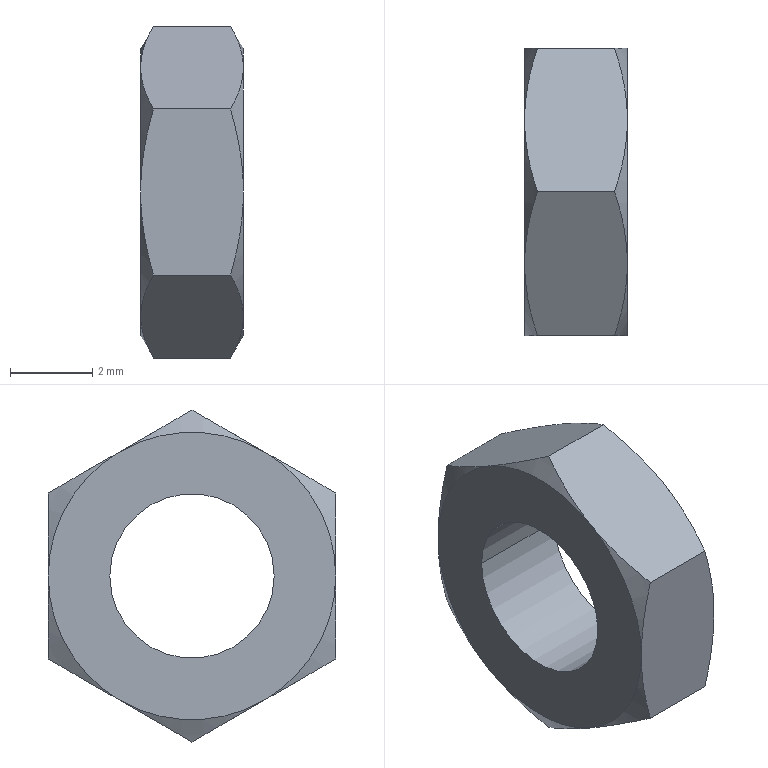Component | SolidWorks | MI10x10U(0)+()-1_MI10-M4x0_7 - Nut-2 | 1 solid | 22 faces | box 2.5 x 7 x 8.08 mm | volume 74 mm3 | cone 12 | plane 8 | cylinder 2 | commonest cylinder face diameters 4 x2
build123d program:
from build123d import *

# Parameters (mm, degrees)
SKETCH2_W                        = 14
SKETCH2_H                        = 14
CUT_EXTRUDE1_DEPTH               = 5
SKETCH1_R                        = 2
M4_THREAD_MAJOR_DIA_RELIEF_DEPTH = 6.902


with BuildPart() as part:
    # Sketch1_2 → Revolve1 (revolve)
    with BuildSketch(Plane.XY, mode=Mode.PRIVATE) as revolve1_sk:
        Polygon((0, 0), (0, 3.5), (0.4041, 4.2), (2.096, 4.2), (2.5, 3.5), (2.5, 0), align=None)
    revolve(revolve1_sk.sketch.rotate(Axis((2.5, 0, 0), (-1, 0, 0)), 270), axis=Axis((2.5, 0, 0), (-1, 0, 0)))

    # Sketch2 → Cut-Extrude1 (cut)
    with BuildSketch(Plane(origin=(0, 0, 0), x_dir=(0, 0, -1), z_dir=(1, 0, 0))):
        Rectangle(SKETCH2_W, SKETCH2_H)
        Polygon((-3.5, -2.021), (0, -4.041), (3.5, -2.021), (3.5, 2.021), (0, 4.041), (-3.5, 2.021), align=None, mode=Mode.SUBTRACT)
    extrude(amount=CUT_EXTRUDE1_DEPTH, mode=Mode.SUBTRACT)

    # Sketch3 → Cut-Revolve1 (revolve, cut)
    with BuildSketch(Plane.XY, mode=Mode.PRIVATE) as cut_revolve1_sk:
        Polygon((0, 0), (0, 2), (0.379, 1.621), (2.121, 1.621), (2.5, 2), (2.5, 0), align=None)
    revolve(cut_revolve1_sk.sketch.rotate(Axis((2.5, 0, 0), (-1, 0, 0)), 270), axis=Axis((2.5, 0, 0), (-1, 0, 0)), mode=Mode.SUBTRACT)

    # Sketch1 → M4 thread major-dia relief (cut, through all)
    with BuildSketch(Plane.ZY):
        Circle(SKETCH1_R)
    extrude(amount=-M4_THREAD_MAJOR_DIA_RELIEF_DEPTH, mode=Mode.SUBTRACT)


solid = part.part

# Placed as in the assembly
solid = solid.moved(Location((-0.994, 30.452, 72.77), (90, 0, 0)))
STEP:
#1=COLOUR_RGB('',0.7922,0.8196,0.9333);
#2=FILL_AREA_STYLE_COLOUR('',#1);
#3=FILL_AREA_STYLE('',(#2));
#4=SURFACE_STYLE_FILL_AREA(#3);
#5=SURFACE_SIDE_STYLE('',(#4));
#6=SURFACE_STYLE_USAGE(.BOTH.,#5);
#7=PRESENTATION_STYLE_ASSIGNMENT((#6));
#8=CARTESIAN_POINT('',(-0.03913,1.12,2.865));
#9=VERTEX_POINT('',#8);
#10=CARTESIAN_POINT('',(-0.03913,1.278,2.865));
#11=VERTEX_POINT('',#10);
#12=CARTESIAN_POINT('',(-0.03913,1.199,2.865));
#13=DIRECTION('',(1.,-0.,-0.));
#14=DIRECTION('',(0.,1.,0.));
#15=AXIS2_PLACEMENT_3D('',#12,#13,#14);
#16=CIRCLE('',#15,0.07874);
#17=EDGE_CURVE('',#9,#11,#16,.T.);
#18=ORIENTED_EDGE('',*,*,#17,.F.);
#19=CARTESIAN_POINT('',(0.05929,1.12,2.865));
#20=VERTEX_POINT('',#19);
#21=CARTESIAN_POINT('',(-0.03913,1.12,2.865));
#22=DIRECTION('',(1.,-0.,-0.));
#23=VECTOR('',#22,39.37);
#24=LINE('',#21,#23);
#25=EDGE_CURVE('',#9,#20,#24,.T.);
#26=ORIENTED_EDGE('',*,*,#25,.T.);
#27=CARTESIAN_POINT('',(0.05929,1.278,2.865));
#28=VERTEX_POINT('',#27);
#29=CARTESIAN_POINT('',(0.05929,1.199,2.865));
#30=DIRECTION('',(1.,-0.,-0.));
#31=DIRECTION('',(0.,1.,0.));
#32=AXIS2_PLACEMENT_3D('',#29,#30,#31);
#33=CIRCLE('',#32,0.07874);
#34=EDGE_CURVE('',#20,#28,#33,.T.);
#35=ORIENTED_EDGE('',*,*,#34,.T.);
#36=CARTESIAN_POINT('',(-0.03913,1.278,2.865));
#37=DIRECTION('',(1.,-0.,-0.));
#38=VECTOR('',#37,39.37);
#39=LINE('',#36,#38);
#40=EDGE_CURVE('',#11,#28,#39,.T.);
#41=ORIENTED_EDGE('',*,*,#40,.F.);
#42=EDGE_LOOP('',(#18,#26,#35,#41));
#43=FACE_OUTER_BOUND('',#42,.T.);
#44=CARTESIAN_POINT('',(-0.03913,1.199,2.865));
#45=DIRECTION('',(1.,-0.,-0.));
#46=DIRECTION('',(0.,1.,0.));
#47=AXIS2_PLACEMENT_3D('',#44,#45,#46);
#48=CYLINDRICAL_SURFACE('',#47,0.07874);
#49=ADVANCED_FACE('',(#43),#48,.F.);
#50=CARTESIAN_POINT('',(0.05929,1.061,2.865));
#51=VERTEX_POINT('',#50);
#52=CARTESIAN_POINT('',(0.04698,1.061,2.785));
#53=VERTEX_POINT('',#52);
#54=CARTESIAN_POINT('',(0.05929,1.061,2.865));
#55=CARTESIAN_POINT('',(0.05929,1.061,2.852));
#56=CARTESIAN_POINT('',(0.05814,1.061,2.838));
#57=CARTESIAN_POINT('',(0.05385,1.061,2.812));
#58=CARTESIAN_POINT('',(0.05072,1.061,2.798));
#59=CARTESIAN_POINT('',(0.04698,1.061,2.785));
#60=B_SPLINE_CURVE_WITH_KNOTS('',3,(#54,#55,#56,#57,#58,#59),.UNSPECIFIED.,.F.,.F.,(4,2,4),(0.01092,0.01194,0.01297),.UNSPECIFIED.);
#61=EDGE_CURVE('',#51,#53,#60,.T.);
#62=ORIENTED_EDGE('',*,*,#61,.T.);
#63=CARTESIAN_POINT('',(0.05929,1.13,2.746));
#64=VERTEX_POINT('',#63);
#65=CARTESIAN_POINT('',(0.04698,1.061,2.785));
#66=CARTESIAN_POINT('',(0.0545,1.084,2.772));
#67=CARTESIAN_POINT('',(0.05929,1.107,2.759));
#68=CARTESIAN_POINT('',(0.05929,1.13,2.746));
#69=B_SPLINE_CURVE_WITH_KNOTS('',3,(#65,#66,#67,#68),.UNSPECIFIED.,.F.,.F.,(4,4),(0.00000024,0.002045),.UNSPECIFIED.);
#70=EDGE_CURVE('',#53,#64,#69,.T.);
#71=ORIENTED_EDGE('',*,*,#70,.T.);
#72=CARTESIAN_POINT('',(0.05929,1.199,2.865));
#73=DIRECTION('',(1.,-0.,-0.));
#74=DIRECTION('',(0.,1.,0.));
#75=AXIS2_PLACEMENT_3D('',#72,#73,#74);
#76=CIRCLE('',#75,0.1378);
#77=EDGE_CURVE('',#51,#64,#76,.T.);
#78=ORIENTED_EDGE('',*,*,#77,.F.);
#79=EDGE_LOOP('',(#62,#71,#78));
#80=FACE_OUTER_BOUND('',#79,.T.);
#81=CARTESIAN_POINT('',(0.04338,1.199,2.865));
#82=DIRECTION('',(-1.,0.,0.));
#83=DIRECTION('',(-0.,-1.,0.));
#84=AXIS2_PLACEMENT_3D('',#81,#82,#83);
#85=CONICAL_SURFACE('',#84,0.1654,1.047);
#86=ADVANCED_FACE('',(#80),#85,.T.);
#87=CARTESIAN_POINT('',(0.05929,1.268,2.746));
#88=VERTEX_POINT('',#87);
#89=CARTESIAN_POINT('',(0.05929,1.199,2.865));
#90=DIRECTION('',(1.,-0.,-0.));
#91=DIRECTION('',(0.,1.,0.));
#92=AXIS2_PLACEMENT_3D('',#89,#90,#91);
#93=CIRCLE('',#92,0.1378);
#94=EDGE_CURVE('',#64,#88,#93,.T.);
#95=ORIENTED_EDGE('',*,*,#94,.F.);
#96=CARTESIAN_POINT('',(0.04698,1.199,2.706));
#97=VERTEX_POINT('',#96);
#98=CARTESIAN_POINT('',(0.05929,1.13,2.746));
#99=CARTESIAN_POINT('',(0.05929,1.142,2.739));
#100=CARTESIAN_POINT('',(0.05811,1.153,2.732));
#101=CARTESIAN_POINT('',(0.05382,1.176,2.719));
#102=CARTESIAN_POINT('',(0.05073,1.188,2.712));
#103=CARTESIAN_POINT('',(0.04698,1.199,2.706));
#104=B_SPLINE_CURVE_WITH_KNOTS('',3,(#98,#99,#100,#101,#102,#103),.UNSPECIFIED.,.F.,.F.,(4,2,4),(0.002045,0.003063,0.004082),.UNSPECIFIED.);
#105=EDGE_CURVE('',#64,#97,#104,.T.);
#106=ORIENTED_EDGE('',*,*,#105,.T.);
#107=CARTESIAN_POINT('',(0.04698,1.199,2.706));
#108=CARTESIAN_POINT('',(0.0545,1.221,2.719));
#109=CARTESIAN_POINT('',(0.05929,1.244,2.732));
#110=CARTESIAN_POINT('',(0.05929,1.268,2.746));
#111=B_SPLINE_CURVE_WITH_KNOTS('',3,(#107,#108,#109,#110),.UNSPECIFIED.,.F.,.F.,(4,4),(0.00000024,0.002045),.UNSPECIFIED.);
#112=EDGE_CURVE('',#97,#88,#111,.T.);
#113=ORIENTED_EDGE('',*,*,#112,.T.);
#114=EDGE_LOOP('',(#95,#106,#113));
#115=FACE_OUTER_BOUND('',#114,.T.);
#116=CARTESIAN_POINT('',(0.04338,1.199,2.865));
#117=DIRECTION('',(-1.,0.,0.));
#118=DIRECTION('',(-0.,-1.,0.));
#119=AXIS2_PLACEMENT_3D('',#116,#117,#118);
#120=CONICAL_SURFACE('',#119,0.1654,1.047);
#121=ADVANCED_FACE('',(#115),#120,.T.);
#122=CARTESIAN_POINT('',(0.05929,1.337,2.865));
#123=VERTEX_POINT('',#122);
#124=CARTESIAN_POINT('',(0.05929,1.199,2.865));
#125=DIRECTION('',(1.,-0.,-0.));
#126=DIRECTION('',(0.,1.,0.));
#127=AXIS2_PLACEMENT_3D('',#124,#125,#126);
#128=CIRCLE('',#127,0.1378);
#129=EDGE_CURVE('',#88,#123,#128,.T.);
#130=ORIENTED_EDGE('',*,*,#129,.F.);
#131=CARTESIAN_POINT('',(0.04698,1.337,2.785));
#132=VERTEX_POINT('',#131);
#133=CARTESIAN_POINT('',(0.05929,1.268,2.746));
#134=CARTESIAN_POINT('',(0.05929,1.28,2.752));
#135=CARTESIAN_POINT('',(0.05811,1.291,2.759));
#136=CARTESIAN_POINT('',(0.05382,1.314,2.772));
#137=CARTESIAN_POINT('',(0.05073,1.325,2.779));
#138=CARTESIAN_POINT('',(0.04698,1.337,2.785));
#139=B_SPLINE_CURVE_WITH_KNOTS('',3,(#133,#134,#135,#136,#137,#138),.UNSPECIFIED.,.F.,.F.,(4,2,4),(0.002045,0.003063,0.004082),.UNSPECIFIED.);
#140=EDGE_CURVE('',#88,#132,#139,.T.);
#141=ORIENTED_EDGE('',*,*,#140,.T.);
#142=CARTESIAN_POINT('',(0.04698,1.337,2.785));
#143=CARTESIAN_POINT('',(0.05072,1.337,2.798));
#144=CARTESIAN_POINT('',(0.05385,1.337,2.812));
#145=CARTESIAN_POINT('',(0.05814,1.337,2.838));
#146=CARTESIAN_POINT('',(0.05929,1.337,2.852));
#147=CARTESIAN_POINT('',(0.05929,1.337,2.865));
#148=B_SPLINE_CURVE_WITH_KNOTS('',3,(#142,#143,#144,#145,#146,#147),.UNSPECIFIED.,.F.,.F.,(4,2,4),(0.003619,0.004642,0.005664),.UNSPECIFIED.);
#149=EDGE_CURVE('',#132,#123,#148,.T.);
#150=ORIENTED_EDGE('',*,*,#149,.T.);
#151=EDGE_LOOP('',(#130,#141,#150));
#152=FACE_OUTER_BOUND('',#151,.T.);
#153=CARTESIAN_POINT('',(0.04338,1.199,2.865));
#154=DIRECTION('',(-1.,0.,0.));
#155=DIRECTION('',(-0.,-1.,0.));
#156=AXIS2_PLACEMENT_3D('',#153,#154,#155);
#157=CONICAL_SURFACE('',#156,0.1654,1.047);
#158=ADVANCED_FACE('',(#152),#157,.T.);
#159=CARTESIAN_POINT('',(0.05929,1.13,2.984));
#160=VERTEX_POINT('',#159);
#161=CARTESIAN_POINT('',(0.04698,1.061,2.945));
#162=VERTEX_POINT('',#161);
#163=CARTESIAN_POINT('',(0.05929,1.13,2.984));
#164=CARTESIAN_POINT('',(0.05929,1.118,2.978));
#165=CARTESIAN_POINT('',(0.05811,1.107,2.971));
#166=CARTESIAN_POINT('',(0.05382,1.084,2.958));
#167=CARTESIAN_POINT('',(0.05073,1.072,2.951));
#168=CARTESIAN_POINT('',(0.04698,1.061,2.945));
#169=B_SPLINE_CURVE_WITH_KNOTS('',3,(#163,#164,#165,#166,#167,#168),.UNSPECIFIED.,.F.,.F.,(4,2,4),(0.002045,0.003063,0.004082),.UNSPECIFIED.);
#170=EDGE_CURVE('',#160,#162,#169,.T.);
#171=ORIENTED_EDGE('',*,*,#170,.T.);
#172=CARTESIAN_POINT('',(0.04698,1.061,2.945));
#173=CARTESIAN_POINT('',(0.0507,1.061,2.932));
#174=CARTESIAN_POINT('',(0.05379,1.061,2.919));
#175=CARTESIAN_POINT('',(0.0581,1.061,2.892));
#176=CARTESIAN_POINT('',(0.05929,1.061,2.878));
#177=CARTESIAN_POINT('',(0.05929,1.061,2.865));
#178=B_SPLINE_CURVE_WITH_KNOTS('',3,(#172,#173,#174,#175,#176,#177),.UNSPECIFIED.,.F.,.F.,(4,2,4),(0.008871,0.009895,0.01092),.UNSPECIFIED.);
#179=EDGE_CURVE('',#162,#51,#178,.T.);
#180=ORIENTED_EDGE('',*,*,#179,.T.);
#181=CARTESIAN_POINT('',(0.05929,1.199,2.865));
#182=DIRECTION('',(1.,-0.,-0.));
#183=DIRECTION('',(0.,1.,0.));
#184=AXIS2_PLACEMENT_3D('',#181,#182,#183);
#185=CIRCLE('',#184,0.1378);
#186=EDGE_CURVE('',#160,#51,#185,.T.);
#187=ORIENTED_EDGE('',*,*,#186,.F.);
#188=EDGE_LOOP('',(#171,#180,#187));
#189=FACE_OUTER_BOUND('',#188,.T.);
#190=CARTESIAN_POINT('',(0.04338,1.199,2.865));
#191=DIRECTION('',(-1.,0.,0.));
#192=DIRECTION('',(-0.,-1.,0.));
#193=AXIS2_PLACEMENT_3D('',#190,#191,#192);
#194=CONICAL_SURFACE('',#193,0.1654,1.047);
#195=ADVANCED_FACE('',(#189),#194,.T.);
#196=CARTESIAN_POINT('',(0.05929,1.268,2.984));
#197=VERTEX_POINT('',#196);
#198=CARTESIAN_POINT('',(0.05929,1.199,2.865));
#199=DIRECTION('',(1.,-0.,-0.));
#200=DIRECTION('',(0.,1.,0.));
#201=AXIS2_PLACEMENT_3D('',#198,#199,#200);
#202=CIRCLE('',#201,0.1378);
#203=EDGE_CURVE('',#123,#197,#202,.T.);
#204=ORIENTED_EDGE('',*,*,#203,.F.);
#205=CARTESIAN_POINT('',(0.04698,1.337,2.945));
#206=VERTEX_POINT('',#205);
#207=CARTESIAN_POINT('',(0.05929,1.337,2.865));
#208=CARTESIAN_POINT('',(0.05929,1.337,2.878));
#209=CARTESIAN_POINT('',(0.0581,1.337,2.892));
#210=CARTESIAN_POINT('',(0.05379,1.337,2.919));
#211=CARTESIAN_POINT('',(0.0507,1.337,2.932));
#212=CARTESIAN_POINT('',(0.04698,1.337,2.945));
#213=B_SPLINE_CURVE_WITH_KNOTS('',3,(#207,#208,#209,#210,#211,#212),.UNSPECIFIED.,.F.,.F.,(4,2,4),(0.005664,0.006687,0.007709),.UNSPECIFIED.);
#214=EDGE_CURVE('',#123,#206,#213,.T.);
#215=ORIENTED_EDGE('',*,*,#214,.T.);
#216=CARTESIAN_POINT('',(0.04698,1.337,2.945));
#217=CARTESIAN_POINT('',(0.0545,1.314,2.958));
#218=CARTESIAN_POINT('',(0.05929,1.291,2.971));
#219=CARTESIAN_POINT('',(0.05929,1.268,2.984));
#220=B_SPLINE_CURVE_WITH_KNOTS('',3,(#216,#217,#218,#219),.UNSPECIFIED.,.F.,.F.,(4,4),(0.00000024,0.002045),.UNSPECIFIED.);
#221=EDGE_CURVE('',#206,#197,#220,.T.);
#222=ORIENTED_EDGE('',*,*,#221,.T.);
#223=EDGE_LOOP('',(#204,#215,#222));
#224=FACE_OUTER_BOUND('',#223,.T.);
#225=CARTESIAN_POINT('',(0.04338,1.199,2.865));
#226=DIRECTION('',(-1.,0.,0.));
#227=DIRECTION('',(-0.,-1.,0.));
#228=AXIS2_PLACEMENT_3D('',#225,#226,#227);
#229=CONICAL_SURFACE('',#228,0.1654,1.047);
#230=ADVANCED_FACE('',(#224),#229,.T.);
#231=CARTESIAN_POINT('',(0.05929,1.199,2.865));
#232=DIRECTION('',(1.,-0.,-0.));
#233=DIRECTION('',(0.,1.,0.));
#234=AXIS2_PLACEMENT_3D('',#231,#232,#233);
#235=CIRCLE('',#234,0.07874);
#236=EDGE_CURVE('',#28,#20,#235,.T.);
#237=ORIENTED_EDGE('',*,*,#236,.F.);
#238=ORIENTED_EDGE('',*,*,#34,.F.);
#239=EDGE_LOOP('',(#237,#238));
#240=FACE_BOUND('',#239,.T.);
#241=ORIENTED_EDGE('',*,*,#203,.T.);
#242=CARTESIAN_POINT('',(0.05929,1.199,2.865));
#243=DIRECTION('',(1.,-0.,-0.));
#244=DIRECTION('',(0.,1.,0.));
#245=AXIS2_PLACEMENT_3D('',#242,#243,#244);
#246=CIRCLE('',#245,0.1378);
#247=EDGE_CURVE('',#197,#160,#246,.T.);
#248=ORIENTED_EDGE('',*,*,#247,.T.);
#249=ORIENTED_EDGE('',*,*,#186,.T.);
#250=ORIENTED_EDGE('',*,*,#77,.T.);
#251=ORIENTED_EDGE('',*,*,#94,.T.);
#252=ORIENTED_EDGE('',*,*,#129,.T.);
#253=EDGE_LOOP('',(#241,#248,#249,#250,#251,#252));
#254=FACE_OUTER_BOUND('',#253,.T.);
#255=CARTESIAN_POINT('',(0.05929,1.199,2.865));
#256=DIRECTION('',(-1.,0.,0.));
#257=DIRECTION('',(-0.,-1.,-0.));
#258=AXIS2_PLACEMENT_3D('',#255,#256,#257);
#259=PLANE('',#258);
#260=ADVANCED_FACE('',(#240,#254),#259,.F.);
#261=CARTESIAN_POINT('',(0.04698,1.199,3.024));
#262=VERTEX_POINT('',#261);
#263=CARTESIAN_POINT('',(0.05929,1.268,2.984));
#264=CARTESIAN_POINT('',(0.05929,1.256,2.991));
#265=CARTESIAN_POINT('',(0.05811,1.244,2.998));
#266=CARTESIAN_POINT('',(0.05382,1.221,3.011));
#267=CARTESIAN_POINT('',(0.05073,1.21,3.018));
#268=CARTESIAN_POINT('',(0.04698,1.199,3.024));
#269=B_SPLINE_CURVE_WITH_KNOTS('',3,(#263,#264,#265,#266,#267,#268),.UNSPECIFIED.,.F.,.F.,(4,2,4),(0.002045,0.003063,0.004082),.UNSPECIFIED.);
#270=EDGE_CURVE('',#197,#262,#269,.T.);
#271=ORIENTED_EDGE('',*,*,#270,.T.);
#272=CARTESIAN_POINT('',(0.04698,1.199,3.024));
#273=CARTESIAN_POINT('',(0.0545,1.176,3.011));
#274=CARTESIAN_POINT('',(0.05929,1.153,2.998));
#275=CARTESIAN_POINT('',(0.05929,1.13,2.984));
#276=B_SPLINE_CURVE_WITH_KNOTS('',3,(#272,#273,#274,#275),.UNSPECIFIED.,.F.,.F.,(4,4),(0.00000024,0.002045),.UNSPECIFIED.);
#277=EDGE_CURVE('',#262,#160,#276,.T.);
#278=ORIENTED_EDGE('',*,*,#277,.T.);
#279=ORIENTED_EDGE('',*,*,#247,.F.);
#280=EDGE_LOOP('',(#271,#278,#279));
#281=FACE_OUTER_BOUND('',#280,.T.);
#282=CARTESIAN_POINT('',(0.04338,1.199,2.865));
#283=DIRECTION('',(-1.,0.,0.));
#284=DIRECTION('',(-0.,-1.,0.));
#285=AXIS2_PLACEMENT_3D('',#282,#283,#284);
#286=CONICAL_SURFACE('',#285,0.1654,1.047);
#287=ADVANCED_FACE('',(#281),#286,.T.);
#288=CARTESIAN_POINT('',(-0.02683,1.337,2.785));
#289=VERTEX_POINT('',#288);
#290=CARTESIAN_POINT('',(-0.1376,1.337,2.785));
#291=DIRECTION('',(1.,-0.,-0.));
#292=VECTOR('',#291,39.37);
#293=LINE('',#290,#292);
#294=EDGE_CURVE('',#289,#132,#293,.T.);
#295=ORIENTED_EDGE('',*,*,#294,.F.);
#296=CARTESIAN_POINT('',(-0.03913,1.337,2.865));
#297=VERTEX_POINT('',#296);
#298=CARTESIAN_POINT('',(-0.03913,1.337,2.865));
#299=CARTESIAN_POINT('',(-0.03913,1.337,2.852));
#300=CARTESIAN_POINT('',(-0.03798,1.337,2.838));
#301=CARTESIAN_POINT('',(-0.0337,1.337,2.812));
#302=CARTESIAN_POINT('',(-0.03056,1.337,2.798));
#303=CARTESIAN_POINT('',(-0.02683,1.337,2.785));
#304=B_SPLINE_CURVE_WITH_KNOTS('',3,(#298,#299,#300,#301,#302,#303),.UNSPECIFIED.,.F.,.F.,(4,2,4),(0.01092,0.01194,0.01297),.UNSPECIFIED.);
#305=EDGE_CURVE('',#297,#289,#304,.T.);
#306=ORIENTED_EDGE('',*,*,#305,.F.);
#307=CARTESIAN_POINT('',(-0.02683,1.337,2.945));
#308=VERTEX_POINT('',#307);
#309=CARTESIAN_POINT('',(-0.02683,1.337,2.945));
#310=CARTESIAN_POINT('',(-0.03054,1.337,2.932));
#311=CARTESIAN_POINT('',(-0.03363,1.337,2.919));
#312=CARTESIAN_POINT('',(-0.03795,1.337,2.892));
#313=CARTESIAN_POINT('',(-0.03913,1.337,2.878));
#314=CARTESIAN_POINT('',(-0.03913,1.337,2.865));
#315=B_SPLINE_CURVE_WITH_KNOTS('',3,(#309,#310,#311,#312,#313,#314),.UNSPECIFIED.,.F.,.F.,(4,2,4),(0.008871,0.009895,0.01092),.UNSPECIFIED.);
#316=EDGE_CURVE('',#308,#297,#315,.T.);
#317=ORIENTED_EDGE('',*,*,#316,.F.);
#318=CARTESIAN_POINT('',(-0.1376,1.337,2.945));
#319=DIRECTION('',(1.,-0.,-0.));
#320=VECTOR('',#319,39.37);
#321=LINE('',#318,#320);
#322=EDGE_CURVE('',#308,#206,#321,.T.);
#323=ORIENTED_EDGE('',*,*,#322,.T.);
#324=ORIENTED_EDGE('',*,*,#214,.F.);
#325=ORIENTED_EDGE('',*,*,#149,.F.);
#326=EDGE_LOOP('',(#295,#306,#317,#323,#324,#325));
#327=FACE_OUTER_BOUND('',#326,.T.);
#328=CARTESIAN_POINT('',(-0.1376,1.337,2.945));
#329=DIRECTION('',(-0.,-1.,-0.));
#330=DIRECTION('',(1.,-0.,-0.));
#331=AXIS2_PLACEMENT_3D('',#328,#329,#330);
#332=PLANE('',#331);
#333=ADVANCED_FACE('',(#327),#332,.F.);
#334=CARTESIAN_POINT('',(-0.02683,1.199,2.706));
#335=VERTEX_POINT('',#334);
#336=CARTESIAN_POINT('',(-0.1376,1.199,2.706));
#337=DIRECTION('',(1.,-0.,-0.));
#338=VECTOR('',#337,39.37);
#339=LINE('',#336,#338);
#340=EDGE_CURVE('',#335,#97,#339,.T.);
#341=ORIENTED_EDGE('',*,*,#340,.F.);
#342=CARTESIAN_POINT('',(-0.03913,1.268,2.746));
#343=VERTEX_POINT('',#342);
#344=CARTESIAN_POINT('',(-0.03913,1.268,2.746));
#345=CARTESIAN_POINT('',(-0.03913,1.256,2.739));
#346=CARTESIAN_POINT('',(-0.03796,1.244,2.732));
#347=CARTESIAN_POINT('',(-0.03367,1.221,2.719));
#348=CARTESIAN_POINT('',(-0.03057,1.21,2.712));
#349=CARTESIAN_POINT('',(-0.02683,1.199,2.706));
#350=B_SPLINE_CURVE_WITH_KNOTS('',3,(#344,#345,#346,#347,#348,#349),.UNSPECIFIED.,.F.,.F.,(4,2,4),(0.002045,0.003063,0.004082),.UNSPECIFIED.);
#351=EDGE_CURVE('',#343,#335,#350,.T.);
#352=ORIENTED_EDGE('',*,*,#351,.F.);
#353=CARTESIAN_POINT('',(-0.02683,1.337,2.785));
#354=CARTESIAN_POINT('',(-0.03434,1.314,2.772));
#355=CARTESIAN_POINT('',(-0.03913,1.291,2.759));
#356=CARTESIAN_POINT('',(-0.03913,1.268,2.746));
#357=B_SPLINE_CURVE_WITH_KNOTS('',3,(#353,#354,#355,#356),.UNSPECIFIED.,.F.,.F.,(4,4),(0.00000024,0.002045),.UNSPECIFIED.);
#358=EDGE_CURVE('',#289,#343,#357,.T.);
#359=ORIENTED_EDGE('',*,*,#358,.F.);
#360=ORIENTED_EDGE('',*,*,#294,.T.);
#361=ORIENTED_EDGE('',*,*,#140,.F.);
#362=ORIENTED_EDGE('',*,*,#112,.F.);
#363=EDGE_LOOP('',(#341,#352,#359,#360,#361,#362));
#364=FACE_OUTER_BOUND('',#363,.T.);
#365=CARTESIAN_POINT('',(-0.1376,1.337,2.785));
#366=DIRECTION('',(0.,-0.5,0.866));
#367=DIRECTION('',(0.,0.866,0.5));
#368=AXIS2_PLACEMENT_3D('',#365,#366,#367);
#369=PLANE('',#368);
#370=ADVANCED_FACE('',(#364),#369,.F.);
#371=CARTESIAN_POINT('',(-0.02683,1.061,2.785));
#372=VERTEX_POINT('',#371);
#373=CARTESIAN_POINT('',(-0.1376,1.061,2.785));
#374=DIRECTION('',(1.,-0.,-0.));
#375=VECTOR('',#374,39.37);
#376=LINE('',#373,#375);
#377=EDGE_CURVE('',#372,#53,#376,.T.);
#378=ORIENTED_EDGE('',*,*,#377,.F.);
#379=CARTESIAN_POINT('',(-0.03913,1.13,2.746));
#380=VERTEX_POINT('',#379);
#381=CARTESIAN_POINT('',(-0.03913,1.13,2.746));
#382=CARTESIAN_POINT('',(-0.03913,1.118,2.752));
#383=CARTESIAN_POINT('',(-0.03796,1.107,2.759));
#384=CARTESIAN_POINT('',(-0.03367,1.084,2.772));
#385=CARTESIAN_POINT('',(-0.03057,1.072,2.779));
#386=CARTESIAN_POINT('',(-0.02683,1.061,2.785));
#387=B_SPLINE_CURVE_WITH_KNOTS('',3,(#381,#382,#383,#384,#385,#386),.UNSPECIFIED.,.F.,.F.,(4,2,4),(0.002045,0.003063,0.004082),.UNSPECIFIED.);
#388=EDGE_CURVE('',#380,#372,#387,.T.);
#389=ORIENTED_EDGE('',*,*,#388,.F.);
#390=CARTESIAN_POINT('',(-0.02683,1.199,2.706));
#391=CARTESIAN_POINT('',(-0.03434,1.176,2.719));
#392=CARTESIAN_POINT('',(-0.03913,1.153,2.732));
#393=CARTESIAN_POINT('',(-0.03913,1.13,2.746));
#394=B_SPLINE_CURVE_WITH_KNOTS('',3,(#390,#391,#392,#393),.UNSPECIFIED.,.F.,.F.,(4,4),(0.00000024,0.002045),.UNSPECIFIED.);
#395=EDGE_CURVE('',#335,#380,#394,.T.);
#396=ORIENTED_EDGE('',*,*,#395,.F.);
#397=ORIENTED_EDGE('',*,*,#340,.T.);
#398=ORIENTED_EDGE('',*,*,#105,.F.);
#399=ORIENTED_EDGE('',*,*,#70,.F.);
#400=EDGE_LOOP('',(#378,#389,#396,#397,#398,#399));
#401=FACE_OUTER_BOUND('',#400,.T.);
#402=CARTESIAN_POINT('',(-0.1376,1.199,2.706));
#403=DIRECTION('',(0.,0.5,0.866));
#404=DIRECTION('',(0.,0.866,-0.5));
#405=AXIS2_PLACEMENT_3D('',#402,#403,#404);
#406=PLANE('',#405);
#407=ADVANCED_FACE('',(#401),#406,.F.);
#408=CARTESIAN_POINT('',(-0.02683,1.061,2.945));
#409=VERTEX_POINT('',#408);
#410=CARTESIAN_POINT('',(-0.1376,1.061,2.945));
#411=DIRECTION('',(1.,-0.,-0.));
#412=VECTOR('',#411,39.37);
#413=LINE('',#410,#412);
#414=EDGE_CURVE('',#409,#162,#413,.T.);
#415=ORIENTED_EDGE('',*,*,#414,.F.);
#416=CARTESIAN_POINT('',(-0.03913,1.061,2.865));
#417=VERTEX_POINT('',#416);
#418=CARTESIAN_POINT('',(-0.03913,1.061,2.865));
#419=CARTESIAN_POINT('',(-0.03913,1.061,2.878));
#420=CARTESIAN_POINT('',(-0.03795,1.061,2.892));
#421=CARTESIAN_POINT('',(-0.03363,1.061,2.919));
#422=CARTESIAN_POINT('',(-0.03054,1.061,2.932));
#423=CARTESIAN_POINT('',(-0.02683,1.061,2.945));
#424=B_SPLINE_CURVE_WITH_KNOTS('',3,(#418,#419,#420,#421,#422,#423),.UNSPECIFIED.,.F.,.F.,(4,2,4),(0.005664,0.006687,0.007709),.UNSPECIFIED.);
#425=EDGE_CURVE('',#417,#409,#424,.T.);
#426=ORIENTED_EDGE('',*,*,#425,.F.);
#427=CARTESIAN_POINT('',(-0.02683,1.061,2.785));
#428=CARTESIAN_POINT('',(-0.03056,1.061,2.798));
#429=CARTESIAN_POINT('',(-0.0337,1.061,2.812));
#430=CARTESIAN_POINT('',(-0.03798,1.061,2.838));
#431=CARTESIAN_POINT('',(-0.03913,1.061,2.852));
#432=CARTESIAN_POINT('',(-0.03913,1.061,2.865));
#433=B_SPLINE_CURVE_WITH_KNOTS('',3,(#427,#428,#429,#430,#431,#432),.UNSPECIFIED.,.F.,.F.,(4,2,4),(0.003619,0.004642,0.005664),.UNSPECIFIED.);
#434=EDGE_CURVE('',#372,#417,#433,.T.);
#435=ORIENTED_EDGE('',*,*,#434,.F.);
#436=ORIENTED_EDGE('',*,*,#377,.T.);
#437=ORIENTED_EDGE('',*,*,#61,.F.);
#438=ORIENTED_EDGE('',*,*,#179,.F.);
#439=EDGE_LOOP('',(#415,#426,#435,#436,#437,#438));
#440=FACE_OUTER_BOUND('',#439,.T.);
#441=CARTESIAN_POINT('',(-0.1376,1.061,2.785));
#442=DIRECTION('',(0.,1.,0.));
#443=DIRECTION('',(-1.,0.,0.));
#444=AXIS2_PLACEMENT_3D('',#441,#442,#443);
#445=PLANE('',#444);
#446=ADVANCED_FACE('',(#440),#445,.F.);
#447=CARTESIAN_POINT('',(-0.02683,1.199,3.024));
#448=VERTEX_POINT('',#447);
#449=CARTESIAN_POINT('',(-0.1376,1.199,3.024));
#450=DIRECTION('',(1.,-0.,-0.));
#451=VECTOR('',#450,39.37);
#452=LINE('',#449,#451);
#453=EDGE_CURVE('',#448,#262,#452,.T.);
#454=ORIENTED_EDGE('',*,*,#453,.F.);
#455=CARTESIAN_POINT('',(-0.03913,1.13,2.984));
#456=VERTEX_POINT('',#455);
#457=CARTESIAN_POINT('',(-0.03913,1.13,2.984));
#458=CARTESIAN_POINT('',(-0.03913,1.142,2.991));
#459=CARTESIAN_POINT('',(-0.03796,1.153,2.998));
#460=CARTESIAN_POINT('',(-0.03367,1.176,3.011));
#461=CARTESIAN_POINT('',(-0.03057,1.188,3.018));
#462=CARTESIAN_POINT('',(-0.02683,1.199,3.024));
#463=B_SPLINE_CURVE_WITH_KNOTS('',3,(#457,#458,#459,#460,#461,#462),.UNSPECIFIED.,.F.,.F.,(4,2,4),(0.002045,0.003063,0.004082),.UNSPECIFIED.);
#464=EDGE_CURVE('',#456,#448,#463,.T.);
#465=ORIENTED_EDGE('',*,*,#464,.F.);
#466=CARTESIAN_POINT('',(-0.02683,1.061,2.945));
#467=CARTESIAN_POINT('',(-0.03434,1.084,2.958));
#468=CARTESIAN_POINT('',(-0.03913,1.107,2.971));
#469=CARTESIAN_POINT('',(-0.03913,1.13,2.984));
#470=B_SPLINE_CURVE_WITH_KNOTS('',3,(#466,#467,#468,#469),.UNSPECIFIED.,.F.,.F.,(4,4),(0.00000024,0.002045),.UNSPECIFIED.);
#471=EDGE_CURVE('',#409,#456,#470,.T.);
#472=ORIENTED_EDGE('',*,*,#471,.F.);
#473=ORIENTED_EDGE('',*,*,#414,.T.);
#474=ORIENTED_EDGE('',*,*,#170,.F.);
#475=ORIENTED_EDGE('',*,*,#277,.F.);
#476=EDGE_LOOP('',(#454,#465,#472,#473,#474,#475));
#477=FACE_OUTER_BOUND('',#476,.T.);
#478=CARTESIAN_POINT('',(-0.1376,1.061,2.945));
#479=DIRECTION('',(-0.,0.5,-0.866));
#480=DIRECTION('',(-0.,-0.866,-0.5));
#481=AXIS2_PLACEMENT_3D('',#478,#479,#480);
#482=PLANE('',#481);
#483=ADVANCED_FACE('',(#477),#482,.F.);
#484=ORIENTED_EDGE('',*,*,#322,.F.);
#485=CARTESIAN_POINT('',(-0.03913,1.268,2.984));
#486=VERTEX_POINT('',#485);
#487=CARTESIAN_POINT('',(-0.03913,1.268,2.984));
#488=CARTESIAN_POINT('',(-0.03913,1.28,2.978));
#489=CARTESIAN_POINT('',(-0.03796,1.291,2.971));
#490=CARTESIAN_POINT('',(-0.03367,1.314,2.958));
#491=CARTESIAN_POINT('',(-0.03057,1.325,2.951));
#492=CARTESIAN_POINT('',(-0.02683,1.337,2.945));
#493=B_SPLINE_CURVE_WITH_KNOTS('',3,(#487,#488,#489,#490,#491,#492),.UNSPECIFIED.,.F.,.F.,(4,2,4),(0.002045,0.003063,0.004082),.UNSPECIFIED.);
#494=EDGE_CURVE('',#486,#308,#493,.T.);
#495=ORIENTED_EDGE('',*,*,#494,.F.);
#496=CARTESIAN_POINT('',(-0.02683,1.199,3.024));
#497=CARTESIAN_POINT('',(-0.03434,1.221,3.011));
#498=CARTESIAN_POINT('',(-0.03913,1.244,2.998));
#499=CARTESIAN_POINT('',(-0.03913,1.268,2.984));
#500=B_SPLINE_CURVE_WITH_KNOTS('',3,(#496,#497,#498,#499),.UNSPECIFIED.,.F.,.F.,(4,4),(0.00000024,0.002045),.UNSPECIFIED.);
#501=EDGE_CURVE('',#448,#486,#500,.T.);
#502=ORIENTED_EDGE('',*,*,#501,.F.);
#503=ORIENTED_EDGE('',*,*,#453,.T.);
#504=ORIENTED_EDGE('',*,*,#270,.F.);
#505=ORIENTED_EDGE('',*,*,#221,.F.);
#506=EDGE_LOOP('',(#484,#495,#502,#503,#504,#505));
#507=FACE_OUTER_BOUND('',#506,.T.);
#508=CARTESIAN_POINT('',(-0.1376,1.199,3.024));
#509=DIRECTION('',(-0.,-0.5,-0.866));
#510=DIRECTION('',(-0.,-0.866,0.5));
#511=AXIS2_PLACEMENT_3D('',#508,#509,#510);
#512=PLANE('',#511);
#513=ADVANCED_FACE('',(#507),#512,.F.);
#514=CARTESIAN_POINT('',(-0.03913,1.199,2.865));
#515=DIRECTION('',(1.,-0.,-0.));
#516=DIRECTION('',(0.,1.,0.));
#517=AXIS2_PLACEMENT_3D('',#514,#515,#516);
#518=CIRCLE('',#517,0.1378);
#519=EDGE_CURVE('',#486,#456,#518,.T.);
#520=ORIENTED_EDGE('',*,*,#519,.T.);
#521=ORIENTED_EDGE('',*,*,#464,.T.);
#522=ORIENTED_EDGE('',*,*,#501,.T.);
#523=EDGE_LOOP('',(#520,#521,#522));
#524=FACE_OUTER_BOUND('',#523,.T.);
#525=CARTESIAN_POINT('',(-0.03913,1.199,2.865));
#526=DIRECTION('',(1.,-0.,-0.));
#527=DIRECTION('',(0.,1.,0.));
#528=AXIS2_PLACEMENT_3D('',#525,#526,#527);
#529=CONICAL_SURFACE('',#528,0.1378,1.047);
#530=ADVANCED_FACE('',(#524),#529,.T.);
#531=CARTESIAN_POINT('',(-0.03913,1.199,2.865));
#532=DIRECTION('',(1.,-0.,-0.));
#533=DIRECTION('',(0.,1.,0.));
#534=AXIS2_PLACEMENT_3D('',#531,#532,#533);
#535=CIRCLE('',#534,0.1378);
#536=EDGE_CURVE('',#456,#417,#535,.T.);
#537=ORIENTED_EDGE('',*,*,#536,.T.);
#538=ORIENTED_EDGE('',*,*,#425,.T.);
#539=ORIENTED_EDGE('',*,*,#471,.T.);
#540=EDGE_LOOP('',(#537,#538,#539));
#541=FACE_OUTER_BOUND('',#540,.T.);
#542=CARTESIAN_POINT('',(-0.03913,1.199,2.865));
#543=DIRECTION('',(1.,-0.,-0.));
#544=DIRECTION('',(0.,1.,0.));
#545=AXIS2_PLACEMENT_3D('',#542,#543,#544);
#546=CONICAL_SURFACE('',#545,0.1378,1.047);
#547=ADVANCED_FACE('',(#541),#546,.T.);
#548=CARTESIAN_POINT('',(-0.03913,1.199,2.865));
#549=DIRECTION('',(1.,-0.,-0.));
#550=DIRECTION('',(0.,1.,0.));
#551=AXIS2_PLACEMENT_3D('',#548,#549,#550);
#552=CIRCLE('',#551,0.1378);
#553=EDGE_CURVE('',#417,#380,#552,.T.);
#554=ORIENTED_EDGE('',*,*,#553,.T.);
#555=ORIENTED_EDGE('',*,*,#388,.T.);
#556=ORIENTED_EDGE('',*,*,#434,.T.);
#557=EDGE_LOOP('',(#554,#555,#556));
#558=FACE_OUTER_BOUND('',#557,.T.);
#559=CARTESIAN_POINT('',(-0.03913,1.199,2.865));
#560=DIRECTION('',(1.,-0.,-0.));
#561=DIRECTION('',(0.,1.,0.));
#562=AXIS2_PLACEMENT_3D('',#559,#560,#561);
#563=CONICAL_SURFACE('',#562,0.1378,1.047);
#564=ADVANCED_FACE('',(#558),#563,.T.);
#565=CARTESIAN_POINT('',(-0.03913,1.199,2.865));
#566=DIRECTION('',(1.,-0.,-0.));
#567=DIRECTION('',(0.,1.,0.));
#568=AXIS2_PLACEMENT_3D('',#565,#566,#567);
#569=CIRCLE('',#568,0.1378);
#570=EDGE_CURVE('',#380,#343,#569,.T.);
#571=ORIENTED_EDGE('',*,*,#570,.T.);
#572=ORIENTED_EDGE('',*,*,#351,.T.);
#573=ORIENTED_EDGE('',*,*,#395,.T.);
#574=EDGE_LOOP('',(#571,#572,#573));
#575=FACE_OUTER_BOUND('',#574,.T.);
#576=CARTESIAN_POINT('',(-0.03913,1.199,2.865));
#577=DIRECTION('',(1.,-0.,-0.));
#578=DIRECTION('',(0.,1.,0.));
#579=AXIS2_PLACEMENT_3D('',#576,#577,#578);
#580=CONICAL_SURFACE('',#579,0.1378,1.047);
#581=ADVANCED_FACE('',(#575),#580,.T.);
#582=CARTESIAN_POINT('',(-0.03913,1.199,2.865));
#583=DIRECTION('',(1.,-0.,-0.));
#584=DIRECTION('',(0.,1.,0.));
#585=AXIS2_PLACEMENT_3D('',#582,#583,#584);
#586=CIRCLE('',#585,0.1378);
#587=EDGE_CURVE('',#343,#297,#586,.T.);
#588=ORIENTED_EDGE('',*,*,#587,.T.);
#589=ORIENTED_EDGE('',*,*,#305,.T.);
#590=ORIENTED_EDGE('',*,*,#358,.T.);
#591=EDGE_LOOP('',(#588,#589,#590));
#592=FACE_OUTER_BOUND('',#591,.T.);
#593=CARTESIAN_POINT('',(-0.03913,1.199,2.865));
#594=DIRECTION('',(1.,-0.,-0.));
#595=DIRECTION('',(0.,1.,0.));
#596=AXIS2_PLACEMENT_3D('',#593,#594,#595);
#597=CONICAL_SURFACE('',#596,0.1378,1.047);
#598=ADVANCED_FACE('',(#592),#597,.T.);
#599=CARTESIAN_POINT('',(-0.03913,1.199,2.865));
#600=DIRECTION('',(1.,-0.,-0.));
#601=DIRECTION('',(0.,1.,0.));
#602=AXIS2_PLACEMENT_3D('',#599,#600,#601);
#603=CIRCLE('',#602,0.07874);
#604=EDGE_CURVE('',#11,#9,#603,.T.);
#605=ORIENTED_EDGE('',*,*,#604,.T.);
#606=ORIENTED_EDGE('',*,*,#17,.T.);
#607=EDGE_LOOP('',(#605,#606));
#608=FACE_BOUND('',#607,.T.);
#609=CARTESIAN_POINT('',(-0.03913,1.199,2.865));
#610=DIRECTION('',(1.,-0.,-0.));
#611=DIRECTION('',(0.,1.,0.));
#612=AXIS2_PLACEMENT_3D('',#609,#610,#611);
#613=CIRCLE('',#612,0.1378);
#614=EDGE_CURVE('',#297,#486,#613,.T.);
#615=ORIENTED_EDGE('',*,*,#614,.F.);
#616=ORIENTED_EDGE('',*,*,#587,.F.);
#617=ORIENTED_EDGE('',*,*,#570,.F.);
#618=ORIENTED_EDGE('',*,*,#553,.F.);
#619=ORIENTED_EDGE('',*,*,#536,.F.);
#620=ORIENTED_EDGE('',*,*,#519,.F.);
#621=EDGE_LOOP('',(#615,#616,#617,#618,#619,#620));
#622=FACE_OUTER_BOUND('',#621,.T.);
#623=CARTESIAN_POINT('',(-0.03913,1.199,3.003));
#624=DIRECTION('',(1.,-0.,-0.));
#625=DIRECTION('',(0.,1.,0.));
#626=AXIS2_PLACEMENT_3D('',#623,#624,#625);
#627=PLANE('',#626);
#628=ADVANCED_FACE('',(#608,#622),#627,.F.);
#629=ORIENTED_EDGE('',*,*,#494,.T.);
#630=ORIENTED_EDGE('',*,*,#316,.T.);
#631=ORIENTED_EDGE('',*,*,#614,.T.);
#632=EDGE_LOOP('',(#629,#630,#631));
#633=FACE_OUTER_BOUND('',#632,.T.);
#634=CARTESIAN_POINT('',(-0.03913,1.199,2.865));
#635=DIRECTION('',(1.,-0.,-0.));
#636=DIRECTION('',(0.,1.,0.));
#637=AXIS2_PLACEMENT_3D('',#634,#635,#636);
#638=CONICAL_SURFACE('',#637,0.1378,1.047);
#639=ADVANCED_FACE('',(#633),#638,.T.);
#640=ORIENTED_EDGE('',*,*,#25,.F.);
#641=ORIENTED_EDGE('',*,*,#604,.F.);
#642=ORIENTED_EDGE('',*,*,#40,.T.);
#643=ORIENTED_EDGE('',*,*,#236,.T.);
#644=EDGE_LOOP('',(#640,#641,#642,#643));
#645=FACE_OUTER_BOUND('',#644,.T.);
#646=CARTESIAN_POINT('',(-0.03913,1.199,2.865));
#647=DIRECTION('',(1.,-0.,-0.));
#648=DIRECTION('',(0.,1.,0.));
#649=AXIS2_PLACEMENT_3D('',#646,#647,#648);
#650=CYLINDRICAL_SURFACE('',#649,0.07874);
#651=ADVANCED_FACE('',(#645),#650,.F.);
#652=CLOSED_SHELL('',(#49,#86,#121,#158,#195,#230,#260,#287,#333,#370,#407,#446,#483,#513,#530,#547,#564,#581,#598,#628,#639,#651));
#653=MANIFOLD_SOLID_BREP('',#652);
#654=STYLED_ITEM('',(#7),#653);
#655=(LENGTH_UNIT()NAMED_UNIT(*)SI_UNIT($,.METRE.));
#656=LENGTH_MEASURE_WITH_UNIT(LENGTH_MEASURE(0.0254),#655);
#657=DIMENSIONAL_EXPONENTS(1.,0.,0.,0.,0.,0.,0.);
#658=(CONVERSION_BASED_UNIT('',#656)LENGTH_UNIT()NAMED_UNIT(#657));
#659=UNCERTAINTY_MEASURE_WITH_UNIT(LENGTH_MEASURE(0.00001),#658,'','');
#660=(NAMED_UNIT(*)PLANE_ANGLE_UNIT()SI_UNIT($,.RADIAN.));
#661=(NAMED_UNIT(*)SI_UNIT($,.STERADIAN.)SOLID_ANGLE_UNIT());
#662=(GEOMETRIC_REPRESENTATION_CONTEXT(3)GLOBAL_UNCERTAINTY_ASSIGNED_CONTEXT((#659))GLOBAL_UNIT_ASSIGNED_CONTEXT((#658,#660,#661))REPRESENTATION_CONTEXT('',''));
#663=MECHANICAL_DESIGN_GEOMETRIC_PRESENTATION_REPRESENTATION('',(#654),#662);
#664=PRESENTATION_LAYER_ASSIGNMENT('','',(#654));
#665=CARTESIAN_POINT('',(0.,0.,0.));
#666=DIRECTION('',(0.,0.,1.));
#667=DIRECTION('',(1.,0.,0.));
#668=AXIS2_PLACEMENT_3D('',#665,#666,#667);
#669=(LENGTH_UNIT()NAMED_UNIT(*)SI_UNIT($,.METRE.));
#670=LENGTH_MEASURE_WITH_UNIT(LENGTH_MEASURE(0.0254),#669);
#671=DIMENSIONAL_EXPONENTS(1.,0.,0.,0.,0.,0.,0.);
#672=(CONVERSION_BASED_UNIT('',#670)LENGTH_UNIT()NAMED_UNIT(#671));
#673=UNCERTAINTY_MEASURE_WITH_UNIT(LENGTH_MEASURE(0.00001),#672,'','');
#674=(NAMED_UNIT(*)PLANE_ANGLE_UNIT()SI_UNIT($,.RADIAN.));
#675=(NAMED_UNIT(*)SI_UNIT($,.STERADIAN.)SOLID_ANGLE_UNIT());
#676=(GEOMETRIC_REPRESENTATION_CONTEXT(3)GLOBAL_UNCERTAINTY_ASSIGNED_CONTEXT((#673))GLOBAL_UNIT_ASSIGNED_CONTEXT((#672,#674,#675))REPRESENTATION_CONTEXT('',''));
#677=ADVANCED_BREP_SHAPE_REPRESENTATION('',(#653,#668),#676);